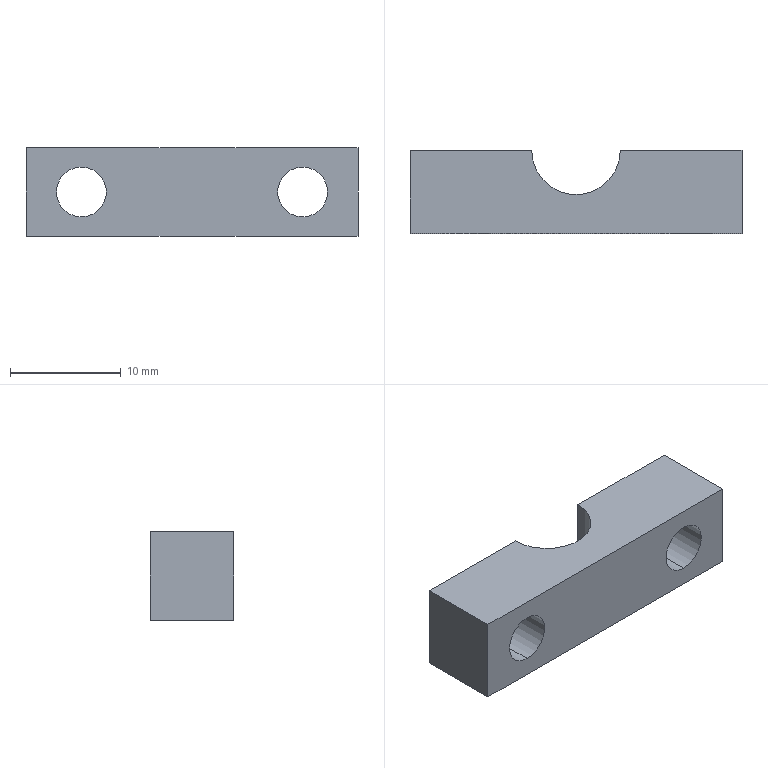Component | SolidWorks | JL001-05-02-1_JL001-05-01-013-1 | 1 solid | 12 faces | box 30 x 7.5 x 8 mm | volume 1360 mm3 | plane 7 | cylinder 5 | commonest cylinder face diameters 4.5 x4 8 x1
build123d program:
from build123d import *

# Parameters (mm, degrees)
SKETCH1_W                      = 30
SKETCH1_H                      = 8
BOSS_EXTRUDE1_DEPTH            = 7.5
F_4_5_4_5_DIAMETER_HOLE1_D     = 4.5
F_4_5_4_5_DIAMETER_HOLE1_DEPTH = 10.1
F_4_5_4_5_DIAMETER_HOLE1_TIP   = 1.352
F_8_0_8_DIAMETER_HOLE1_D       = 8
F_8_0_8_DIAMETER_HOLE1_DEPTH   = 10.1
F_8_0_8_DIAMETER_HOLE1_TIP     = 2.403


with BuildPart() as part:
    # Sketch1 → Boss-Extrude1 (new body)
    with BuildSketch(Plane(origin=(0, 0, 0), x_dir=(1, 0, 0), z_dir=(0, 1, 0))):
        Rectangle(SKETCH1_W, SKETCH1_H)
    extrude(amount=BOSS_EXTRUDE1_DEPTH)

    # 4.5 _4.5_ Diameter Hole1
    with Locations(Plane(origin=(0, 7.5, 0), x_dir=(1, 0, 0), z_dir=(0, 1, 0))):
        with Locations((-10, 0), (10, 0)):
            Hole(F_4_5_4_5_DIAMETER_HOLE1_D / 2, depth=F_4_5_4_5_DIAMETER_HOLE1_DEPTH)
            with Locations((0, 0, -(F_4_5_4_5_DIAMETER_HOLE1_DEPTH + F_4_5_4_5_DIAMETER_HOLE1_TIP / 2))):  # 118° drill point
                Cone(0, F_4_5_4_5_DIAMETER_HOLE1_D / 2, F_4_5_4_5_DIAMETER_HOLE1_TIP, mode=Mode.SUBTRACT)

    # 8.0 _8_ Diameter Hole1
    with Locations(Plane.XY.offset(4)):
        with Locations((0, 0)):
            Hole(F_8_0_8_DIAMETER_HOLE1_D / 2, depth=F_8_0_8_DIAMETER_HOLE1_DEPTH)
            with Locations((0, 0, -(F_8_0_8_DIAMETER_HOLE1_DEPTH + F_8_0_8_DIAMETER_HOLE1_TIP / 2))):  # 118° drill point
                Cone(0, F_8_0_8_DIAMETER_HOLE1_D / 2, F_8_0_8_DIAMETER_HOLE1_TIP, mode=Mode.SUBTRACT)


solid = part.part

# Placed as in the assembly
solid = solid.moved(Location((0, 1047.5, 94), (180, 0, 0)))
STEP:
#1=COLOUR_RGB('',0.7922,0.8196,0.9333);
#2=FILL_AREA_STYLE_COLOUR('',#1);
#3=FILL_AREA_STYLE('',(#2));
#4=SURFACE_STYLE_FILL_AREA(#3);
#5=SURFACE_SIDE_STYLE('',(#4));
#6=SURFACE_STYLE_USAGE(.BOTH.,#5);
#7=PRESENTATION_STYLE_ASSIGNMENT((#6));
#8=CARTESIAN_POINT('',(0.3937,41.24,3.612));
#9=VERTEX_POINT('',#8);
#10=CARTESIAN_POINT('',(0.3937,41.24,3.789));
#11=VERTEX_POINT('',#10);
#12=CARTESIAN_POINT('',(0.3937,41.24,3.701));
#13=DIRECTION('',(0.,-1.,0.));
#14=DIRECTION('',(0.,0.,1.));
#15=AXIS2_PLACEMENT_3D('',#12,#13,#14);
#16=CIRCLE('',#15,0.08858);
#17=EDGE_CURVE('',#9,#11,#16,.T.);
#18=ORIENTED_EDGE('',*,*,#17,.F.);
#19=CARTESIAN_POINT('',(0.3937,40.945,3.612));
#20=VERTEX_POINT('',#19);
#21=CARTESIAN_POINT('',(0.3937,40.945,3.612));
#22=DIRECTION('',(0.,-1.,0.));
#23=VECTOR('',#22,39.37);
#24=LINE('',#21,#23);
#25=EDGE_CURVE('',#9,#20,#24,.T.);
#26=ORIENTED_EDGE('',*,*,#25,.T.);
#27=CARTESIAN_POINT('',(0.3937,40.945,3.789));
#28=VERTEX_POINT('',#27);
#29=CARTESIAN_POINT('',(0.3937,40.945,3.701));
#30=DIRECTION('',(0.,-1.,0.));
#31=DIRECTION('',(0.,0.,1.));
#32=AXIS2_PLACEMENT_3D('',#29,#30,#31);
#33=CIRCLE('',#32,0.08858);
#34=EDGE_CURVE('',#20,#28,#33,.T.);
#35=ORIENTED_EDGE('',*,*,#34,.T.);
#36=CARTESIAN_POINT('',(0.3937,40.945,3.789));
#37=DIRECTION('',(0.,-1.,0.));
#38=VECTOR('',#37,39.37);
#39=LINE('',#36,#38);
#40=EDGE_CURVE('',#11,#28,#39,.T.);
#41=ORIENTED_EDGE('',*,*,#40,.F.);
#42=EDGE_LOOP('',(#18,#26,#35,#41));
#43=FACE_OUTER_BOUND('',#42,.T.);
#44=CARTESIAN_POINT('',(0.3937,40.945,3.701));
#45=DIRECTION('',(0.,-1.,0.));
#46=DIRECTION('',(0.,0.,1.));
#47=AXIS2_PLACEMENT_3D('',#44,#45,#46);
#48=CYLINDRICAL_SURFACE('',#47,0.08858);
#49=ADVANCED_FACE('',(#43),#48,.F.);
#50=CARTESIAN_POINT('',(-0.3937,41.24,3.612));
#51=VERTEX_POINT('',#50);
#52=CARTESIAN_POINT('',(-0.3937,41.24,3.789));
#53=VERTEX_POINT('',#52);
#54=CARTESIAN_POINT('',(-0.3937,41.24,3.701));
#55=DIRECTION('',(0.,-1.,0.));
#56=DIRECTION('',(0.,0.,1.));
#57=AXIS2_PLACEMENT_3D('',#54,#55,#56);
#58=CIRCLE('',#57,0.08858);
#59=EDGE_CURVE('',#51,#53,#58,.T.);
#60=ORIENTED_EDGE('',*,*,#59,.F.);
#61=CARTESIAN_POINT('',(-0.3937,40.945,3.612));
#62=VERTEX_POINT('',#61);
#63=CARTESIAN_POINT('',(-0.3937,40.945,3.612));
#64=DIRECTION('',(0.,-1.,0.));
#65=VECTOR('',#64,39.37);
#66=LINE('',#63,#65);
#67=EDGE_CURVE('',#51,#62,#66,.T.);
#68=ORIENTED_EDGE('',*,*,#67,.T.);
#69=CARTESIAN_POINT('',(-0.3937,40.945,3.789));
#70=VERTEX_POINT('',#69);
#71=CARTESIAN_POINT('',(-0.3937,40.945,3.701));
#72=DIRECTION('',(0.,-1.,0.));
#73=DIRECTION('',(0.,0.,1.));
#74=AXIS2_PLACEMENT_3D('',#71,#72,#73);
#75=CIRCLE('',#74,0.08858);
#76=EDGE_CURVE('',#62,#70,#75,.T.);
#77=ORIENTED_EDGE('',*,*,#76,.T.);
#78=CARTESIAN_POINT('',(-0.3937,40.945,3.789));
#79=DIRECTION('',(0.,-1.,0.));
#80=VECTOR('',#79,39.37);
#81=LINE('',#78,#80);
#82=EDGE_CURVE('',#53,#70,#81,.T.);
#83=ORIENTED_EDGE('',*,*,#82,.F.);
#84=EDGE_LOOP('',(#60,#68,#77,#83));
#85=FACE_OUTER_BOUND('',#84,.T.);
#86=CARTESIAN_POINT('',(-0.3937,40.945,3.701));
#87=DIRECTION('',(0.,-1.,0.));
#88=DIRECTION('',(0.,0.,1.));
#89=AXIS2_PLACEMENT_3D('',#86,#87,#88);
#90=CYLINDRICAL_SURFACE('',#89,0.08858);
#91=ADVANCED_FACE('',(#85),#90,.F.);
#92=CARTESIAN_POINT('',(0.3937,41.24,3.701));
#93=DIRECTION('',(0.,-1.,0.));
#94=DIRECTION('',(0.,0.,1.));
#95=AXIS2_PLACEMENT_3D('',#92,#93,#94);
#96=CIRCLE('',#95,0.08858);
#97=EDGE_CURVE('',#11,#9,#96,.T.);
#98=ORIENTED_EDGE('',*,*,#97,.T.);
#99=ORIENTED_EDGE('',*,*,#17,.T.);
#100=EDGE_LOOP('',(#98,#99));
#101=FACE_BOUND('',#100,.T.);
#102=CARTESIAN_POINT('',(0.1575,41.24,3.543));
#103=VERTEX_POINT('',#102);
#104=CARTESIAN_POINT('',(0.5906,41.24,3.543));
#105=VERTEX_POINT('',#104);
#106=CARTESIAN_POINT('',(0.5906,41.24,3.543));
#107=DIRECTION('',(1.,0.,-0.));
#108=VECTOR('',#107,39.37);
#109=LINE('',#106,#108);
#110=EDGE_CURVE('',#103,#105,#109,.T.);
#111=ORIENTED_EDGE('',*,*,#110,.F.);
#112=CARTESIAN_POINT('',(0.1575,41.24,3.858));
#113=VERTEX_POINT('',#112);
#114=CARTESIAN_POINT('',(0.1575,41.24,3.858));
#115=DIRECTION('',(0.,0.,1.));
#116=VECTOR('',#115,39.37);
#117=LINE('',#114,#116);
#118=EDGE_CURVE('',#103,#113,#117,.T.);
#119=ORIENTED_EDGE('',*,*,#118,.T.);
#120=CARTESIAN_POINT('',(0.5906,41.24,3.858));
#121=VERTEX_POINT('',#120);
#122=CARTESIAN_POINT('',(0.5906,41.24,3.858));
#123=DIRECTION('',(-1.,0.,0.));
#124=VECTOR('',#123,39.37);
#125=LINE('',#122,#124);
#126=EDGE_CURVE('',#121,#113,#125,.T.);
#127=ORIENTED_EDGE('',*,*,#126,.F.);
#128=CARTESIAN_POINT('',(0.5906,41.24,3.543));
#129=DIRECTION('',(0.,0.,1.));
#130=VECTOR('',#129,39.37);
#131=LINE('',#128,#130);
#132=EDGE_CURVE('',#105,#121,#131,.T.);
#133=ORIENTED_EDGE('',*,*,#132,.F.);
#134=EDGE_LOOP('',(#111,#119,#127,#133));
#135=FACE_OUTER_BOUND('',#134,.T.);
#136=CARTESIAN_POINT('',(-0.,41.24,3.701));
#137=DIRECTION('',(0.,-1.,0.));
#138=DIRECTION('',(0.,0.,1.));
#139=AXIS2_PLACEMENT_3D('',#136,#137,#138);
#140=PLANE('',#139);
#141=ADVANCED_FACE('',(#101,#135),#140,.F.);
#142=CARTESIAN_POINT('',(-0.5906,41.24,3.858));
#143=VERTEX_POINT('',#142);
#144=CARTESIAN_POINT('',(-0.5906,41.24,3.543));
#145=VERTEX_POINT('',#144);
#146=CARTESIAN_POINT('',(-0.5906,41.24,3.543));
#147=DIRECTION('',(-0.,0.,-1.));
#148=VECTOR('',#147,39.37);
#149=LINE('',#146,#148);
#150=EDGE_CURVE('',#143,#145,#149,.T.);
#151=ORIENTED_EDGE('',*,*,#150,.T.);
#152=CARTESIAN_POINT('',(-0.5906,40.945,3.543));
#153=VERTEX_POINT('',#152);
#154=CARTESIAN_POINT('',(-0.5906,40.945,3.543));
#155=DIRECTION('',(0.,1.,0.));
#156=VECTOR('',#155,39.37);
#157=LINE('',#154,#156);
#158=EDGE_CURVE('',#153,#145,#157,.T.);
#159=ORIENTED_EDGE('',*,*,#158,.F.);
#160=CARTESIAN_POINT('',(-0.5906,40.945,3.858));
#161=VERTEX_POINT('',#160);
#162=CARTESIAN_POINT('',(-0.5906,40.945,3.543));
#163=DIRECTION('',(-0.,0.,-1.));
#164=VECTOR('',#163,39.37);
#165=LINE('',#162,#164);
#166=EDGE_CURVE('',#161,#153,#165,.T.);
#167=ORIENTED_EDGE('',*,*,#166,.F.);
#168=CARTESIAN_POINT('',(-0.5906,40.945,3.858));
#169=DIRECTION('',(0.,1.,0.));
#170=VECTOR('',#169,39.37);
#171=LINE('',#168,#170);
#172=EDGE_CURVE('',#161,#143,#171,.T.);
#173=ORIENTED_EDGE('',*,*,#172,.T.);
#174=EDGE_LOOP('',(#151,#159,#167,#173));
#175=FACE_OUTER_BOUND('',#174,.T.);
#176=CARTESIAN_POINT('',(-0.5906,40.945,3.543));
#177=DIRECTION('',(1.,0.,-0.));
#178=DIRECTION('',(0.,0.,1.));
#179=AXIS2_PLACEMENT_3D('',#176,#177,#178);
#180=PLANE('',#179);
#181=ADVANCED_FACE('',(#175),#180,.F.);
#182=CARTESIAN_POINT('',(-0.1575,41.24,3.543));
#183=VERTEX_POINT('',#182);
#184=CARTESIAN_POINT('',(0.5906,41.24,3.543));
#185=DIRECTION('',(1.,0.,-0.));
#186=VECTOR('',#185,39.37);
#187=LINE('',#184,#186);
#188=EDGE_CURVE('',#145,#183,#187,.T.);
#189=ORIENTED_EDGE('',*,*,#188,.T.);
#190=CARTESIAN_POINT('',(-0.,41.24,3.543));
#191=DIRECTION('',(0.,0.,1.));
#192=DIRECTION('',(-1.,0.,0.));
#193=AXIS2_PLACEMENT_3D('',#190,#191,#192);
#194=CIRCLE('',#193,0.1575);
#195=EDGE_CURVE('',#183,#103,#194,.T.);
#196=ORIENTED_EDGE('',*,*,#195,.T.);
#197=ORIENTED_EDGE('',*,*,#110,.T.);
#198=CARTESIAN_POINT('',(0.5906,40.945,3.543));
#199=VERTEX_POINT('',#198);
#200=CARTESIAN_POINT('',(0.5906,40.945,3.543));
#201=DIRECTION('',(0.,1.,0.));
#202=VECTOR('',#201,39.37);
#203=LINE('',#200,#202);
#204=EDGE_CURVE('',#199,#105,#203,.T.);
#205=ORIENTED_EDGE('',*,*,#204,.F.);
#206=CARTESIAN_POINT('',(0.5906,40.945,3.543));
#207=DIRECTION('',(1.,0.,-0.));
#208=VECTOR('',#207,39.37);
#209=LINE('',#206,#208);
#210=EDGE_CURVE('',#153,#199,#209,.T.);
#211=ORIENTED_EDGE('',*,*,#210,.F.);
#212=ORIENTED_EDGE('',*,*,#158,.T.);
#213=EDGE_LOOP('',(#189,#196,#197,#205,#211,#212));
#214=FACE_OUTER_BOUND('',#213,.T.);
#215=CARTESIAN_POINT('',(0.5906,40.945,3.543));
#216=DIRECTION('',(0.,0.,1.));
#217=DIRECTION('',(-1.,0.,0.));
#218=AXIS2_PLACEMENT_3D('',#215,#216,#217);
#219=PLANE('',#218);
#220=ADVANCED_FACE('',(#214),#219,.F.);
#221=ORIENTED_EDGE('',*,*,#132,.T.);
#222=CARTESIAN_POINT('',(0.5906,40.945,3.858));
#223=VERTEX_POINT('',#222);
#224=CARTESIAN_POINT('',(0.5906,40.945,3.858));
#225=DIRECTION('',(0.,1.,0.));
#226=VECTOR('',#225,39.37);
#227=LINE('',#224,#226);
#228=EDGE_CURVE('',#223,#121,#227,.T.);
#229=ORIENTED_EDGE('',*,*,#228,.F.);
#230=CARTESIAN_POINT('',(0.5906,40.945,3.543));
#231=DIRECTION('',(0.,0.,1.));
#232=VECTOR('',#231,39.37);
#233=LINE('',#230,#232);
#234=EDGE_CURVE('',#199,#223,#233,.T.);
#235=ORIENTED_EDGE('',*,*,#234,.F.);
#236=ORIENTED_EDGE('',*,*,#204,.T.);
#237=EDGE_LOOP('',(#221,#229,#235,#236));
#238=FACE_OUTER_BOUND('',#237,.T.);
#239=CARTESIAN_POINT('',(0.5906,40.945,3.543));
#240=DIRECTION('',(-1.,0.,0.));
#241=DIRECTION('',(-0.,0.,-1.));
#242=AXIS2_PLACEMENT_3D('',#239,#240,#241);
#243=PLANE('',#242);
#244=ADVANCED_FACE('',(#238),#243,.F.);
#245=ORIENTED_EDGE('',*,*,#126,.T.);
#246=CARTESIAN_POINT('',(-0.1575,41.24,3.858));
#247=VERTEX_POINT('',#246);
#248=CARTESIAN_POINT('',(-0.,41.24,3.858));
#249=DIRECTION('',(0.,0.,1.));
#250=DIRECTION('',(-1.,0.,0.));
#251=AXIS2_PLACEMENT_3D('',#248,#249,#250);
#252=CIRCLE('',#251,0.1575);
#253=EDGE_CURVE('',#247,#113,#252,.T.);
#254=ORIENTED_EDGE('',*,*,#253,.F.);
#255=CARTESIAN_POINT('',(0.5906,41.24,3.858));
#256=DIRECTION('',(-1.,0.,0.));
#257=VECTOR('',#256,39.37);
#258=LINE('',#255,#257);
#259=EDGE_CURVE('',#247,#143,#258,.T.);
#260=ORIENTED_EDGE('',*,*,#259,.T.);
#261=ORIENTED_EDGE('',*,*,#172,.F.);
#262=CARTESIAN_POINT('',(0.5906,40.945,3.858));
#263=DIRECTION('',(-1.,0.,0.));
#264=VECTOR('',#263,39.37);
#265=LINE('',#262,#264);
#266=EDGE_CURVE('',#223,#161,#265,.T.);
#267=ORIENTED_EDGE('',*,*,#266,.F.);
#268=ORIENTED_EDGE('',*,*,#228,.T.);
#269=EDGE_LOOP('',(#245,#254,#260,#261,#267,#268));
#270=FACE_OUTER_BOUND('',#269,.T.);
#271=CARTESIAN_POINT('',(0.5906,40.945,3.858));
#272=DIRECTION('',(-0.,0.,-1.));
#273=DIRECTION('',(1.,0.,-0.));
#274=AXIS2_PLACEMENT_3D('',#271,#272,#273);
#275=PLANE('',#274);
#276=ADVANCED_FACE('',(#270),#275,.F.);
#277=CARTESIAN_POINT('',(0.3937,40.945,3.701));
#278=DIRECTION('',(0.,-1.,0.));
#279=DIRECTION('',(0.,0.,1.));
#280=AXIS2_PLACEMENT_3D('',#277,#278,#279);
#281=CIRCLE('',#280,0.08858);
#282=EDGE_CURVE('',#28,#20,#281,.T.);
#283=ORIENTED_EDGE('',*,*,#282,.F.);
#284=ORIENTED_EDGE('',*,*,#34,.F.);
#285=EDGE_LOOP('',(#283,#284));
#286=FACE_BOUND('',#285,.T.);
#287=CARTESIAN_POINT('',(-0.3937,40.945,3.701));
#288=DIRECTION('',(0.,-1.,0.));
#289=DIRECTION('',(0.,0.,1.));
#290=AXIS2_PLACEMENT_3D('',#287,#288,#289);
#291=CIRCLE('',#290,0.08858);
#292=EDGE_CURVE('',#70,#62,#291,.T.);
#293=ORIENTED_EDGE('',*,*,#292,.F.);
#294=ORIENTED_EDGE('',*,*,#76,.F.);
#295=EDGE_LOOP('',(#293,#294));
#296=FACE_BOUND('',#295,.T.);
#297=ORIENTED_EDGE('',*,*,#166,.T.);
#298=ORIENTED_EDGE('',*,*,#210,.T.);
#299=ORIENTED_EDGE('',*,*,#234,.T.);
#300=ORIENTED_EDGE('',*,*,#266,.T.);
#301=EDGE_LOOP('',(#297,#298,#299,#300));
#302=FACE_OUTER_BOUND('',#301,.T.);
#303=CARTESIAN_POINT('',(-0.,40.945,3.701));
#304=DIRECTION('',(0.,-1.,0.));
#305=DIRECTION('',(0.,0.,1.));
#306=AXIS2_PLACEMENT_3D('',#303,#304,#305);
#307=PLANE('',#306);
#308=ADVANCED_FACE('',(#286,#296,#302),#307,.T.);
#309=CARTESIAN_POINT('',(-0.3937,41.24,3.701));
#310=DIRECTION('',(0.,-1.,0.));
#311=DIRECTION('',(0.,0.,1.));
#312=AXIS2_PLACEMENT_3D('',#309,#310,#311);
#313=CIRCLE('',#312,0.08858);
#314=EDGE_CURVE('',#53,#51,#313,.T.);
#315=ORIENTED_EDGE('',*,*,#314,.T.);
#316=ORIENTED_EDGE('',*,*,#59,.T.);
#317=EDGE_LOOP('',(#315,#316));
#318=FACE_BOUND('',#317,.T.);
#319=ORIENTED_EDGE('',*,*,#259,.F.);
#320=CARTESIAN_POINT('',(-0.1575,41.24,3.858));
#321=DIRECTION('',(-0.,0.,-1.));
#322=VECTOR('',#321,39.37);
#323=LINE('',#320,#322);
#324=EDGE_CURVE('',#247,#183,#323,.T.);
#325=ORIENTED_EDGE('',*,*,#324,.T.);
#326=ORIENTED_EDGE('',*,*,#188,.F.);
#327=ORIENTED_EDGE('',*,*,#150,.F.);
#328=EDGE_LOOP('',(#319,#325,#326,#327));
#329=FACE_OUTER_BOUND('',#328,.T.);
#330=CARTESIAN_POINT('',(-0.,41.24,3.701));
#331=DIRECTION('',(0.,-1.,0.));
#332=DIRECTION('',(0.,0.,1.));
#333=AXIS2_PLACEMENT_3D('',#330,#331,#332);
#334=PLANE('',#333);
#335=ADVANCED_FACE('',(#318,#329),#334,.F.);
#336=ORIENTED_EDGE('',*,*,#67,.F.);
#337=ORIENTED_EDGE('',*,*,#314,.F.);
#338=ORIENTED_EDGE('',*,*,#82,.T.);
#339=ORIENTED_EDGE('',*,*,#292,.T.);
#340=EDGE_LOOP('',(#336,#337,#338,#339));
#341=FACE_OUTER_BOUND('',#340,.T.);
#342=CARTESIAN_POINT('',(-0.3937,40.945,3.701));
#343=DIRECTION('',(0.,-1.,0.));
#344=DIRECTION('',(0.,0.,1.));
#345=AXIS2_PLACEMENT_3D('',#342,#343,#344);
#346=CYLINDRICAL_SURFACE('',#345,0.08858);
#347=ADVANCED_FACE('',(#341),#346,.F.);
#348=ORIENTED_EDGE('',*,*,#25,.F.);
#349=ORIENTED_EDGE('',*,*,#97,.F.);
#350=ORIENTED_EDGE('',*,*,#40,.T.);
#351=ORIENTED_EDGE('',*,*,#282,.T.);
#352=EDGE_LOOP('',(#348,#349,#350,#351));
#353=FACE_OUTER_BOUND('',#352,.T.);
#354=CARTESIAN_POINT('',(0.3937,40.945,3.701));
#355=DIRECTION('',(0.,-1.,0.));
#356=DIRECTION('',(0.,0.,1.));
#357=AXIS2_PLACEMENT_3D('',#354,#355,#356);
#358=CYLINDRICAL_SURFACE('',#357,0.08858);
#359=ADVANCED_FACE('',(#353),#358,.F.);
#360=ORIENTED_EDGE('',*,*,#195,.F.);
#361=ORIENTED_EDGE('',*,*,#324,.F.);
#362=ORIENTED_EDGE('',*,*,#253,.T.);
#363=ORIENTED_EDGE('',*,*,#118,.F.);
#364=EDGE_LOOP('',(#360,#361,#362,#363));
#365=FACE_OUTER_BOUND('',#364,.T.);
#366=CARTESIAN_POINT('',(-0.,41.24,3.858));
#367=DIRECTION('',(0.,0.,1.));
#368=DIRECTION('',(-1.,0.,0.));
#369=AXIS2_PLACEMENT_3D('',#366,#367,#368);
#370=CYLINDRICAL_SURFACE('',#369,0.1575);
#371=ADVANCED_FACE('',(#365),#370,.F.);
#372=CLOSED_SHELL('',(#49,#91,#141,#181,#220,#244,#276,#308,#335,#347,#359,#371));
#373=MANIFOLD_SOLID_BREP('',#372);
#374=STYLED_ITEM('',(#7),#373);
#375=PRESENTATION_LAYER_ASSIGNMENT('','',(#374));
#376=CARTESIAN_POINT('',(0.,0.,0.));
#377=DIRECTION('',(0.,0.,1.));
#378=DIRECTION('',(1.,0.,0.));
#379=AXIS2_PLACEMENT_3D('',#376,#377,#378);
#380=(LENGTH_UNIT()NAMED_UNIT(*)SI_UNIT($,.METRE.));
#381=LENGTH_MEASURE_WITH_UNIT(LENGTH_MEASURE(0.0254),#380);
#382=DIMENSIONAL_EXPONENTS(1.,0.,0.,0.,0.,0.,0.);
#383=(CONVERSION_BASED_UNIT('',#381)LENGTH_UNIT()NAMED_UNIT(#382));
#384=UNCERTAINTY_MEASURE_WITH_UNIT(LENGTH_MEASURE(0.00001),#383,'','');
#385=(NAMED_UNIT(*)PLANE_ANGLE_UNIT()SI_UNIT($,.RADIAN.));
#386=(NAMED_UNIT(*)SI_UNIT($,.STERADIAN.)SOLID_ANGLE_UNIT());
#387=(GEOMETRIC_REPRESENTATION_CONTEXT(3)GLOBAL_UNCERTAINTY_ASSIGNED_CONTEXT((#384))GLOBAL_UNIT_ASSIGNED_CONTEXT((#383,#385,#386))REPRESENTATION_CONTEXT('',''));
#388=ADVANCED_BREP_SHAPE_REPRESENTATION('',(#373,#379),#387);
#389=(LENGTH_UNIT()NAMED_UNIT(*)SI_UNIT($,.METRE.));
#390=LENGTH_MEASURE_WITH_UNIT(LENGTH_MEASURE(0.0254),#389);
#391=DIMENSIONAL_EXPONENTS(1.,0.,0.,0.,0.,0.,0.);
#392=(CONVERSION_BASED_UNIT('',#390)LENGTH_UNIT()NAMED_UNIT(#391));
#393=UNCERTAINTY_MEASURE_WITH_UNIT(LENGTH_MEASURE(0.00001),#392,'','');
#394=(NAMED_UNIT(*)PLANE_ANGLE_UNIT()SI_UNIT($,.RADIAN.));
#395=(NAMED_UNIT(*)SI_UNIT($,.STERADIAN.)SOLID_ANGLE_UNIT());
#396=(GEOMETRIC_REPRESENTATION_CONTEXT(3)GLOBAL_UNCERTAINTY_ASSIGNED_CONTEXT((#393))GLOBAL_UNIT_ASSIGNED_CONTEXT((#392,#394,#395))REPRESENTATION_CONTEXT('',''));
#397=MECHANICAL_DESIGN_GEOMETRIC_PRESENTATION_REPRESENTATION('',(#374),#396);